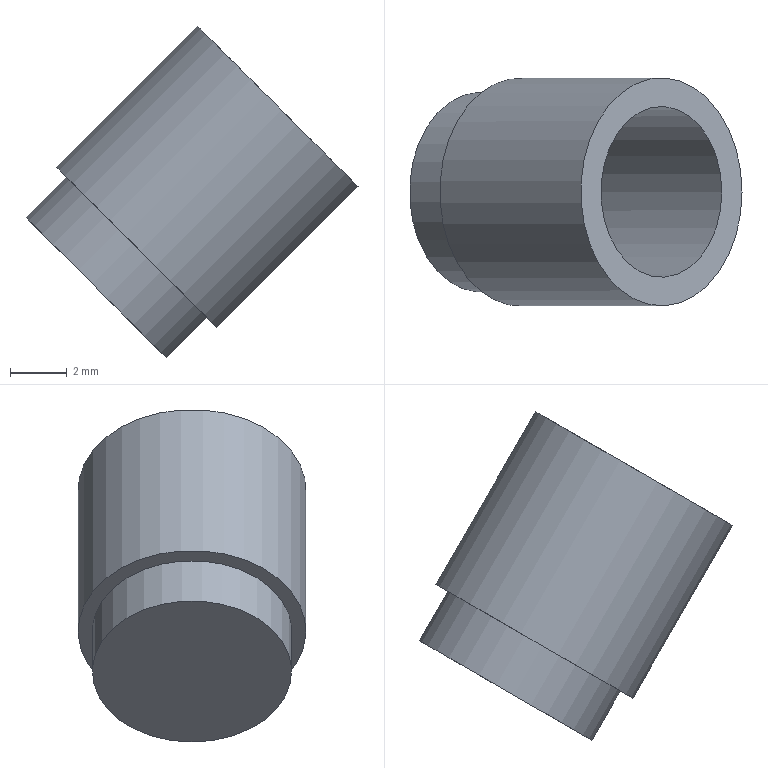Component | NX | VENT_PIPE_CAP | 1 solid | 7 faces | volume 231 mm3 | plane 4 | cylinder 3 | commonest cylinder face diameters 7 x1 8 x1 6 x1